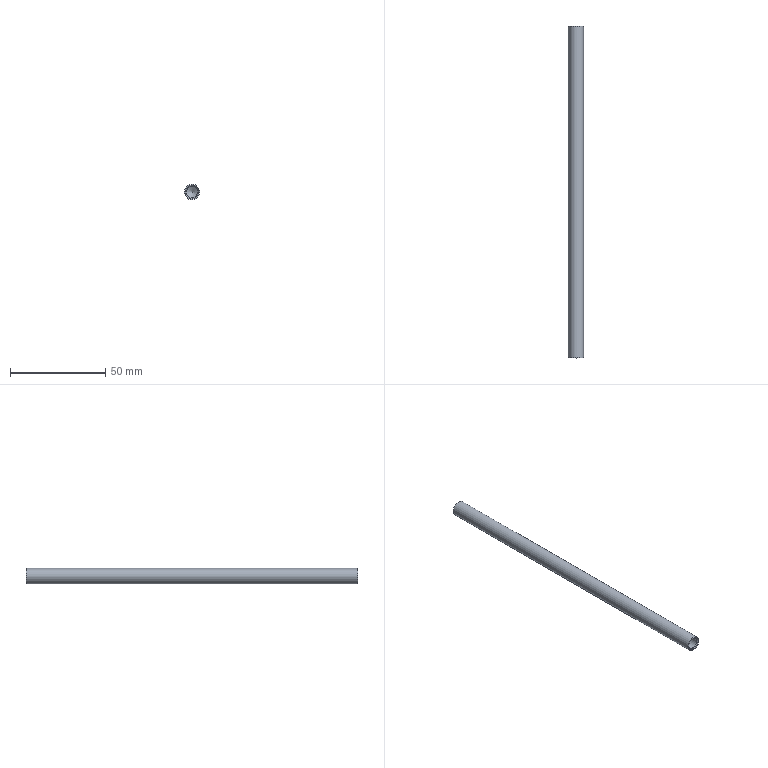Component | NX | CONNECTING_ROD_2 | 1 solid | 9 faces | box 8 x 174 x 8 mm | volume 7746 mm3 | cone 4 | cylinder 3 | plane 2 | commonest cylinder face diameters 6 x2 8 x1
STEP:
#1=CARTESIAN_POINT('',(0.,0.,0.));
#2=DIRECTION('',(0.,0.,1.));
#3=DIRECTION('',(1.,0.,0.));
#4=AXIS2_PLACEMENT_3D('',#1,#2,#3);
#5=CARTESIAN_POINT('',(-245.053,87.,124.782));
#6=VERTEX_POINT('',#5);
#7=CARTESIAN_POINT('',(-248.225,87.,123.303));
#8=DIRECTION('',(0.,-1.,0.));
#9=DIRECTION('',(0.9063,0.,0.4226));
#10=AXIS2_PLACEMENT_3D('',#7,#8,#9);
#11=CIRCLE('',#10,3.5);
#12=CARTESIAN_POINT('',(-248.225,87.,123.303));
#13=DIRECTION('',(0.,1.,0.));
#14=DIRECTION('',(0.9063,0.,0.4226));
#15=AXIS2_PLACEMENT_3D('',#12,#13,#14);
#16=PLANE('',#15);
#17=CARTESIAN_POINT('',(3.5,0.));
#18=CARTESIAN_POINT('',(3.5,-6.062));
#19=CARTESIAN_POINT('',(-1.75,-3.031));
#20=CARTESIAN_POINT('',(-7.,-0.));
#21=CARTESIAN_POINT('',(-1.75,3.031));
#22=CARTESIAN_POINT('',(3.5,6.062));
#23=CARTESIAN_POINT('',(3.5,0.));
#24=(BOUNDED_CURVE()B_SPLINE_CURVE(2,(#17,#18,#19,#20,#21,#22,#23),.UNSPECIFIED.,.T.,.F.)B_SPLINE_CURVE_WITH_KNOTS((1,2,2,2,2,1),(-2.094,0.,2.094,4.189,6.283,8.378),.UNSPECIFIED.)CURVE()GEOMETRIC_REPRESENTATION_ITEM()RATIONAL_B_SPLINE_CURVE((1.,0.5,1.,0.5,1.,0.5,1.))REPRESENTATION_ITEM(''));
#25=(GEOMETRIC_REPRESENTATION_CONTEXT(2)PARAMETRIC_REPRESENTATION_CONTEXT()REPRESENTATION_CONTEXT('',''));
#26=DEFINITIONAL_REPRESENTATION('',(#24),#25);
#27=PCURVE('',#16,#26);
#28=CARTESIAN_POINT('',(-248.225,87.,123.303));
#29=DIRECTION('',(0.,1.,0.));
#30=DIRECTION('',(0.9063,0.,0.4226));
#31=AXIS2_PLACEMENT_3D('',#28,#29,#30);
#32=CONICAL_SURFACE('',#31,3.5,0.7854);
#33=CARTESIAN_POINT('',(6.283,0.));
#34=DIRECTION('',(-1.,0.));
#35=VECTOR('',#34,1.);
#36=LINE('',#33,#35);
#37=(GEOMETRIC_REPRESENTATION_CONTEXT(2)PARAMETRIC_REPRESENTATION_CONTEXT()REPRESENTATION_CONTEXT('',''));
#38=DEFINITIONAL_REPRESENTATION('',(#36),#37);
#39=PCURVE('',#32,#38);
#40=SURFACE_CURVE('',#11,(#27,#39),.PCURVE_S1.);
#41=EDGE_CURVE('',#6,#6,#40,.T.);
#42=ORIENTED_EDGE('',*,*,#41,.T.);
#43=EDGE_LOOP('',(#42));
#44=FACE_BOUND('',#43,.T.);
#45=CARTESIAN_POINT('',(-244.6,87.,124.993));
#46=VERTEX_POINT('',#45);
#47=CARTESIAN_POINT('',(-248.225,87.,123.303));
#48=DIRECTION('',(0.,-1.,0.));
#49=DIRECTION('',(0.9063,0.,0.4226));
#50=AXIS2_PLACEMENT_3D('',#47,#48,#49);
#51=CIRCLE('',#50,4.);
#52=CARTESIAN_POINT('',(4.,-0.));
#53=CARTESIAN_POINT('',(4.,-6.928));
#54=CARTESIAN_POINT('',(-2.,-3.464));
#55=CARTESIAN_POINT('',(-8.,0.));
#56=CARTESIAN_POINT('',(-2.,3.464));
#57=CARTESIAN_POINT('',(4.,6.928));
#58=CARTESIAN_POINT('',(4.,-0.));
#59=(BOUNDED_CURVE()B_SPLINE_CURVE(2,(#52,#53,#54,#55,#56,#57,#58),.UNSPECIFIED.,.T.,.F.)B_SPLINE_CURVE_WITH_KNOTS((1,2,2,2,2,1),(-2.094,0.,2.094,4.189,6.283,8.378),.UNSPECIFIED.)CURVE()GEOMETRIC_REPRESENTATION_ITEM()RATIONAL_B_SPLINE_CURVE((1.,0.5,1.,0.5,1.,0.5,1.))REPRESENTATION_ITEM(''));
#60=(GEOMETRIC_REPRESENTATION_CONTEXT(2)PARAMETRIC_REPRESENTATION_CONTEXT()REPRESENTATION_CONTEXT('',''));
#61=DEFINITIONAL_REPRESENTATION('',(#59),#60);
#62=PCURVE('',#16,#61);
#63=CARTESIAN_POINT('',(-248.225,-87.,123.303));
#64=DIRECTION('',(0.,1.,0.));
#65=DIRECTION('',(0.9063,0.,0.4226));
#66=AXIS2_PLACEMENT_3D('',#63,#64,#65);
#67=CYLINDRICAL_SURFACE('',#66,4.);
#68=CARTESIAN_POINT('',(6.283,174.));
#69=DIRECTION('',(-1.,0.));
#70=VECTOR('',#69,1.);
#71=LINE('',#68,#70);
#72=(GEOMETRIC_REPRESENTATION_CONTEXT(2)PARAMETRIC_REPRESENTATION_CONTEXT()REPRESENTATION_CONTEXT('',''));
#73=DEFINITIONAL_REPRESENTATION('',(#71),#72);
#74=PCURVE('',#67,#73);
#75=SURFACE_CURVE('',#51,(#62,#74),.PCURVE_S1.);
#76=EDGE_CURVE('',#46,#46,#75,.T.);
#77=ORIENTED_EDGE('',*,*,#76,.F.);
#78=EDGE_LOOP('',(#77));
#79=FACE_BOUND('',#78,.T.);
#80=ADVANCED_FACE('',(#44,#79),#16,.T.);
#81=CARTESIAN_POINT('',(-251.397,-87.,121.824));
#82=VERTEX_POINT('',#81);
#83=CARTESIAN_POINT('',(-248.225,-87.,123.303));
#84=DIRECTION('',(0.,1.,0.));
#85=DIRECTION('',(-0.9063,0.,-0.4226));
#86=AXIS2_PLACEMENT_3D('',#83,#84,#85);
#87=CIRCLE('',#86,3.5);
#88=CARTESIAN_POINT('',(-248.225,-87.,123.303));
#89=DIRECTION('',(0.,-1.,0.));
#90=DIRECTION('',(-0.9063,0.,-0.4226));
#91=AXIS2_PLACEMENT_3D('',#88,#89,#90);
#92=PLANE('',#91);
#93=CARTESIAN_POINT('',(3.5,-0.));
#94=CARTESIAN_POINT('',(3.5,-6.062));
#95=CARTESIAN_POINT('',(-1.75,-3.031));
#96=CARTESIAN_POINT('',(-7.,0.));
#97=CARTESIAN_POINT('',(-1.75,3.031));
#98=CARTESIAN_POINT('',(3.5,6.062));
#99=CARTESIAN_POINT('',(3.5,-0.));
#100=(BOUNDED_CURVE()B_SPLINE_CURVE(2,(#93,#94,#95,#96,#97,#98,#99),.UNSPECIFIED.,.T.,.F.)B_SPLINE_CURVE_WITH_KNOTS((1,2,2,2,2,1),(-2.094,0.,2.094,4.189,6.283,8.378),.UNSPECIFIED.)CURVE()GEOMETRIC_REPRESENTATION_ITEM()RATIONAL_B_SPLINE_CURVE((1.,0.5,1.,0.5,1.,0.5,1.))REPRESENTATION_ITEM(''));
#101=(GEOMETRIC_REPRESENTATION_CONTEXT(2)PARAMETRIC_REPRESENTATION_CONTEXT()REPRESENTATION_CONTEXT('',''));
#102=DEFINITIONAL_REPRESENTATION('',(#100),#101);
#103=PCURVE('',#92,#102);
#104=CARTESIAN_POINT('',(-248.225,-87.,123.303));
#105=DIRECTION('',(0.,-1.,0.));
#106=DIRECTION('',(-0.9063,0.,-0.4226));
#107=AXIS2_PLACEMENT_3D('',#104,#105,#106);
#108=CONICAL_SURFACE('',#107,3.5,0.7854);
#109=CARTESIAN_POINT('',(6.283,0.));
#110=DIRECTION('',(-1.,0.));
#111=VECTOR('',#110,1.);
#112=LINE('',#109,#111);
#113=(GEOMETRIC_REPRESENTATION_CONTEXT(2)PARAMETRIC_REPRESENTATION_CONTEXT()REPRESENTATION_CONTEXT('',''));
#114=DEFINITIONAL_REPRESENTATION('',(#112),#113);
#115=PCURVE('',#108,#114);
#116=SURFACE_CURVE('',#87,(#103,#115),.PCURVE_S1.);
#117=EDGE_CURVE('',#82,#82,#116,.T.);
#118=ORIENTED_EDGE('',*,*,#117,.T.);
#119=EDGE_LOOP('',(#118));
#120=FACE_BOUND('',#119,.T.);
#121=CARTESIAN_POINT('',(-244.6,-87.,124.993));
#122=VERTEX_POINT('',#121);
#123=CARTESIAN_POINT('',(-248.225,-87.,123.303));
#124=DIRECTION('',(0.,1.,0.));
#125=DIRECTION('',(0.9063,0.,0.4226));
#126=AXIS2_PLACEMENT_3D('',#123,#124,#125);
#127=CIRCLE('',#126,4.);
#128=CARTESIAN_POINT('',(-4.,-0.));
#129=CARTESIAN_POINT('',(-4.,6.928));
#130=CARTESIAN_POINT('',(2.,3.464));
#131=CARTESIAN_POINT('',(8.,0.));
#132=CARTESIAN_POINT('',(2.,-3.464));
#133=CARTESIAN_POINT('',(-4.,-6.928));
#134=CARTESIAN_POINT('',(-4.,-0.));
#135=(BOUNDED_CURVE()B_SPLINE_CURVE(2,(#128,#129,#130,#131,#132,#133,#134),.UNSPECIFIED.,.T.,.F.)B_SPLINE_CURVE_WITH_KNOTS((1,2,2,2,2,1),(-2.094,0.,2.094,4.189,6.283,8.378),.UNSPECIFIED.)CURVE()GEOMETRIC_REPRESENTATION_ITEM()RATIONAL_B_SPLINE_CURVE((1.,0.5,1.,0.5,1.,0.5,1.))REPRESENTATION_ITEM(''));
#136=(GEOMETRIC_REPRESENTATION_CONTEXT(2)PARAMETRIC_REPRESENTATION_CONTEXT()REPRESENTATION_CONTEXT('',''));
#137=DEFINITIONAL_REPRESENTATION('',(#135),#136);
#138=PCURVE('',#92,#137);
#139=CARTESIAN_POINT('',(0.,0.));
#140=DIRECTION('',(1.,0.));
#141=VECTOR('',#140,1.);
#142=LINE('',#139,#141);
#143=(GEOMETRIC_REPRESENTATION_CONTEXT(2)PARAMETRIC_REPRESENTATION_CONTEXT()REPRESENTATION_CONTEXT('',''));
#144=DEFINITIONAL_REPRESENTATION('',(#142),#143);
#145=PCURVE('',#67,#144);
#146=SURFACE_CURVE('',#127,(#138,#145),.PCURVE_S1.);
#147=EDGE_CURVE('',#122,#122,#146,.T.);
#148=ORIENTED_EDGE('',*,*,#147,.F.);
#149=EDGE_LOOP('',(#148));
#150=FACE_BOUND('',#149,.T.);
#151=ADVANCED_FACE('',(#120,#150),#92,.T.);
#152=ORIENTED_EDGE('',*,*,#76,.T.);
#153=CARTESIAN_POINT('',(-244.6,-87.,124.993));
#154=CARTESIAN_POINT('',(-244.6,87.,124.993));
#155=B_SPLINE_CURVE_WITH_KNOTS('',1,(#153,#154),.UNSPECIFIED.,.F.,.F.,(2,2),(0.,174.),.PIECEWISE_BEZIER_KNOTS.);
#156=CARTESIAN_POINT('',(0.,0.));
#157=DIRECTION('',(0.,1.));
#158=VECTOR('',#157,1.);
#159=LINE('',#156,#158);
#160=(GEOMETRIC_REPRESENTATION_CONTEXT(2)PARAMETRIC_REPRESENTATION_CONTEXT()REPRESENTATION_CONTEXT('',''));
#161=DEFINITIONAL_REPRESENTATION('',(#159),#160);
#162=PCURVE('',#67,#161);
#163=CARTESIAN_POINT('',(6.283,0.));
#164=DIRECTION('',(0.,1.));
#165=VECTOR('',#164,1.);
#166=LINE('',#163,#165);
#167=(GEOMETRIC_REPRESENTATION_CONTEXT(2)PARAMETRIC_REPRESENTATION_CONTEXT()REPRESENTATION_CONTEXT('',''));
#168=DEFINITIONAL_REPRESENTATION('',(#166),#167);
#169=PCURVE('',#67,#168);
#170=SEAM_CURVE('',#155,(#162,#169),.PCURVE_S1.);
#171=EDGE_CURVE('',#122,#46,#170,.T.);
#172=ORIENTED_EDGE('',*,*,#171,.F.);
#173=ORIENTED_EDGE('',*,*,#147,.T.);
#174=ORIENTED_EDGE('',*,*,#171,.T.);
#175=EDGE_LOOP('',(#152,#172,#173,#174));
#176=FACE_BOUND('',#175,.T.);
#177=ADVANCED_FACE('',(#176),#67,.T.);
#178=CARTESIAN_POINT('',(-245.506,70.,124.571));
#179=VERTEX_POINT('',#178);
#180=CARTESIAN_POINT('',(-250.944,70.,122.035));
#181=VERTEX_POINT('',#180);
#182=CARTESIAN_POINT('',(-248.225,70.,123.303));
#183=DIRECTION('',(0.,1.,0.));
#184=DIRECTION('',(-0.9063,0.,-0.4226));
#185=AXIS2_PLACEMENT_3D('',#182,#183,#184);
#186=CIRCLE('',#185,3.);
#187=CARTESIAN_POINT('',(-248.225,70.,123.303));
#188=DIRECTION('',(0.,1.,0.));
#189=DIRECTION('',(0.9063,0.,0.4226));
#190=AXIS2_PLACEMENT_3D('',#187,#188,#189);
#191=CONICAL_SURFACE('',#190,3.,1.03);
#192=CARTESIAN_POINT('',(-3.142,-0.));
#193=DIRECTION('',(1.,0.));
#194=VECTOR('',#193,1.);
#195=LINE('',#192,#194);
#196=(GEOMETRIC_REPRESENTATION_CONTEXT(2)PARAMETRIC_REPRESENTATION_CONTEXT()REPRESENTATION_CONTEXT('',''));
#197=DEFINITIONAL_REPRESENTATION('',(#195),#196);
#198=PCURVE('',#191,#197);
#199=CARTESIAN_POINT('',(-248.225,87.,123.303));
#200=DIRECTION('',(0.,-1.,0.));
#201=DIRECTION('',(-0.9063,0.,-0.4226));
#202=AXIS2_PLACEMENT_3D('',#199,#200,#201);
#203=CYLINDRICAL_SURFACE('',#202,3.);
#204=CARTESIAN_POINT('',(12.566,17.));
#205=DIRECTION('',(-1.,0.));
#206=VECTOR('',#205,1.);
#207=LINE('',#204,#206);
#208=(GEOMETRIC_REPRESENTATION_CONTEXT(2)PARAMETRIC_REPRESENTATION_CONTEXT()REPRESENTATION_CONTEXT('',''));
#209=DEFINITIONAL_REPRESENTATION('',(#207),#208);
#210=PCURVE('',#203,#209);
#211=SURFACE_CURVE('',#186,(#198,#210),.PCURVE_S1.);
#212=EDGE_CURVE('',#179,#181,#211,.T.);
#213=ORIENTED_EDGE('',*,*,#212,.F.);
#214=CARTESIAN_POINT('',(-248.225,68.197,123.303));
#215=VERTEX_POINT('',#214);
#216=CARTESIAN_POINT('',(-248.225,68.197,123.303));
#217=CARTESIAN_POINT('',(-245.506,70.,124.571));
#218=B_SPLINE_CURVE_WITH_KNOTS('',1,(#216,#217),.UNSPECIFIED.,.F.,.F.,(2,2),(-3.5,-0.),.PIECEWISE_BEZIER_KNOTS.);
#219=CARTESIAN_POINT('',(0.,0.));
#220=DIRECTION('',(0.,1.));
#221=VECTOR('',#220,1.);
#222=LINE('',#219,#221);
#223=(GEOMETRIC_REPRESENTATION_CONTEXT(2)PARAMETRIC_REPRESENTATION_CONTEXT()REPRESENTATION_CONTEXT('',''));
#224=DEFINITIONAL_REPRESENTATION('',(#222),#223);
#225=PCURVE('',#191,#224);
#226=CARTESIAN_POINT('',(6.283,0.));
#227=DIRECTION('',(0.,1.));
#228=VECTOR('',#227,1.);
#229=LINE('',#226,#228);
#230=(GEOMETRIC_REPRESENTATION_CONTEXT(2)PARAMETRIC_REPRESENTATION_CONTEXT()REPRESENTATION_CONTEXT('',''));
#231=DEFINITIONAL_REPRESENTATION('',(#229),#230);
#232=PCURVE('',#191,#231);
#233=SEAM_CURVE('',#218,(#225,#232),.PCURVE_S1.);
#234=EDGE_CURVE('',#215,#179,#233,.T.);
#235=ORIENTED_EDGE('',*,*,#234,.F.);
#236=ORIENTED_EDGE('',*,*,#234,.T.);
#237=CARTESIAN_POINT('',(-248.225,70.,123.303));
#238=DIRECTION('',(0.,1.,0.));
#239=DIRECTION('',(-0.9063,0.,-0.4226));
#240=AXIS2_PLACEMENT_3D('',#237,#238,#239);
#241=CIRCLE('',#240,3.);
#242=CARTESIAN_POINT('',(3.142,-0.));
#243=DIRECTION('',(1.,0.));
#244=VECTOR('',#243,1.);
#245=LINE('',#242,#244);
#246=(GEOMETRIC_REPRESENTATION_CONTEXT(2)PARAMETRIC_REPRESENTATION_CONTEXT()REPRESENTATION_CONTEXT('',''));
#247=DEFINITIONAL_REPRESENTATION('',(#245),#246);
#248=PCURVE('',#191,#247);
#249=CARTESIAN_POINT('',(6.283,17.));
#250=DIRECTION('',(-1.,0.));
#251=VECTOR('',#250,1.);
#252=LINE('',#249,#251);
#253=(GEOMETRIC_REPRESENTATION_CONTEXT(2)PARAMETRIC_REPRESENTATION_CONTEXT()REPRESENTATION_CONTEXT('',''));
#254=DEFINITIONAL_REPRESENTATION('',(#252),#253);
#255=PCURVE('',#203,#254);
#256=SURFACE_CURVE('',#241,(#248,#255),.PCURVE_S1.);
#257=EDGE_CURVE('',#181,#179,#256,.T.);
#258=ORIENTED_EDGE('',*,*,#257,.F.);
#259=EDGE_LOOP('',(#213,#235,#236,#258));
#260=FACE_BOUND('',#259,.F.);
#261=ADVANCED_FACE('',(#260),#191,.F.);
#262=CARTESIAN_POINT('',(-245.506,86.5,124.571));
#263=VERTEX_POINT('',#262);
#264=CARTESIAN_POINT('',(-248.225,86.5,123.303));
#265=DIRECTION('',(0.,1.,0.));
#266=DIRECTION('',(0.9063,0.,0.4226));
#267=AXIS2_PLACEMENT_3D('',#264,#265,#266);
#268=CIRCLE('',#267,3.);
#269=CARTESIAN_POINT('',(9.425,0.5));
#270=DIRECTION('',(-1.,0.));
#271=VECTOR('',#270,1.);
#272=LINE('',#269,#271);
#273=(GEOMETRIC_REPRESENTATION_CONTEXT(2)PARAMETRIC_REPRESENTATION_CONTEXT()REPRESENTATION_CONTEXT('',''));
#274=DEFINITIONAL_REPRESENTATION('',(#272),#273);
#275=PCURVE('',#203,#274);
#276=CARTESIAN_POINT('',(0.,-0.5));
#277=DIRECTION('',(1.,0.));
#278=VECTOR('',#277,1.);
#279=LINE('',#276,#278);
#280=(GEOMETRIC_REPRESENTATION_CONTEXT(2)PARAMETRIC_REPRESENTATION_CONTEXT()REPRESENTATION_CONTEXT('',''));
#281=DEFINITIONAL_REPRESENTATION('',(#279),#280);
#282=PCURVE('',#32,#281);
#283=SURFACE_CURVE('',#268,(#275,#282),.PCURVE_S1.);
#284=EDGE_CURVE('',#263,#263,#283,.T.);
#285=ORIENTED_EDGE('',*,*,#284,.F.);
#286=CARTESIAN_POINT('',(-245.506,86.5,124.571));
#287=CARTESIAN_POINT('',(-245.506,70.,124.571));
#288=B_SPLINE_CURVE_WITH_KNOTS('',1,(#286,#287),.UNSPECIFIED.,.F.,.F.,(2,2),(0.5,17.),.PIECEWISE_BEZIER_KNOTS.);
#289=CARTESIAN_POINT('',(9.425,0.));
#290=DIRECTION('',(0.,1.));
#291=VECTOR('',#290,1.);
#292=LINE('',#289,#291);
#293=(GEOMETRIC_REPRESENTATION_CONTEXT(2)PARAMETRIC_REPRESENTATION_CONTEXT()REPRESENTATION_CONTEXT('',''));
#294=DEFINITIONAL_REPRESENTATION('',(#292),#293);
#295=PCURVE('',#203,#294);
#296=CARTESIAN_POINT('',(3.142,0.));
#297=DIRECTION('',(0.,1.));
#298=VECTOR('',#297,1.);
#299=LINE('',#296,#298);
#300=(GEOMETRIC_REPRESENTATION_CONTEXT(2)PARAMETRIC_REPRESENTATION_CONTEXT()REPRESENTATION_CONTEXT('',''));
#301=DEFINITIONAL_REPRESENTATION('',(#299),#300);
#302=PCURVE('',#203,#301);
#303=SEAM_CURVE('',#288,(#295,#302),.PCURVE_S1.);
#304=EDGE_CURVE('',#263,#179,#303,.T.);
#305=ORIENTED_EDGE('',*,*,#304,.T.);
#306=ORIENTED_EDGE('',*,*,#212,.T.);
#307=ORIENTED_EDGE('',*,*,#257,.T.);
#308=ORIENTED_EDGE('',*,*,#304,.F.);
#309=EDGE_LOOP('',(#285,#305,#306,#307,#308));
#310=FACE_BOUND('',#309,.F.);
#311=ADVANCED_FACE('',(#310),#203,.F.);
#312=ORIENTED_EDGE('',*,*,#284,.T.);
#313=CARTESIAN_POINT('',(-245.506,86.5,124.571));
#314=CARTESIAN_POINT('',(-245.053,87.,124.782));
#315=B_SPLINE_CURVE_WITH_KNOTS('',1,(#313,#314),.UNSPECIFIED.,.F.,.F.,(2,2),(-0.7071,0.),.PIECEWISE_BEZIER_KNOTS.);
#316=CARTESIAN_POINT('',(6.283,0.));
#317=DIRECTION('',(0.,1.));
#318=VECTOR('',#317,1.);
#319=LINE('',#316,#318);
#320=(GEOMETRIC_REPRESENTATION_CONTEXT(2)PARAMETRIC_REPRESENTATION_CONTEXT()REPRESENTATION_CONTEXT('',''));
#321=DEFINITIONAL_REPRESENTATION('',(#319),#320);
#322=PCURVE('',#32,#321);
#323=CARTESIAN_POINT('',(0.,0.));
#324=DIRECTION('',(0.,1.));
#325=VECTOR('',#324,1.);
#326=LINE('',#323,#325);
#327=(GEOMETRIC_REPRESENTATION_CONTEXT(2)PARAMETRIC_REPRESENTATION_CONTEXT()REPRESENTATION_CONTEXT('',''));
#328=DEFINITIONAL_REPRESENTATION('',(#326),#327);
#329=PCURVE('',#32,#328);
#330=SEAM_CURVE('',#315,(#322,#329),.PCURVE_S1.);
#331=EDGE_CURVE('',#263,#6,#330,.T.);
#332=ORIENTED_EDGE('',*,*,#331,.T.);
#333=ORIENTED_EDGE('',*,*,#41,.T.);
#334=ORIENTED_EDGE('',*,*,#331,.F.);
#335=EDGE_LOOP('',(#312,#332,#333,#334));
#336=FACE_BOUND('',#335,.F.);
#337=ADVANCED_FACE('',(#336),#32,.F.);
#338=CARTESIAN_POINT('',(-250.944,-70.,122.035));
#339=VERTEX_POINT('',#338);
#340=CARTESIAN_POINT('',(-245.506,-70.,124.571));
#341=VERTEX_POINT('',#340);
#342=CARTESIAN_POINT('',(-248.225,-70.,123.303));
#343=DIRECTION('',(0.,-1.,0.));
#344=DIRECTION('',(0.9063,0.,0.4226));
#345=AXIS2_PLACEMENT_3D('',#342,#343,#344);
#346=CIRCLE('',#345,3.);
#347=CARTESIAN_POINT('',(-248.225,-70.,123.303));
#348=DIRECTION('',(0.,-1.,0.));
#349=DIRECTION('',(-0.9063,0.,-0.4226));
#350=AXIS2_PLACEMENT_3D('',#347,#348,#349);
#351=CONICAL_SURFACE('',#350,3.,1.03);
#352=CARTESIAN_POINT('',(-3.142,0.));
#353=DIRECTION('',(1.,0.));
#354=VECTOR('',#353,1.);
#355=LINE('',#352,#354);
#356=(GEOMETRIC_REPRESENTATION_CONTEXT(2)PARAMETRIC_REPRESENTATION_CONTEXT()REPRESENTATION_CONTEXT('',''));
#357=DEFINITIONAL_REPRESENTATION('',(#355),#356);
#358=PCURVE('',#351,#357);
#359=CARTESIAN_POINT('',(-248.225,-87.,123.303));
#360=DIRECTION('',(0.,1.,0.));
#361=DIRECTION('',(0.9063,0.,0.4226));
#362=AXIS2_PLACEMENT_3D('',#359,#360,#361);
#363=CYLINDRICAL_SURFACE('',#362,3.);
#364=CARTESIAN_POINT('',(12.566,17.));
#365=DIRECTION('',(-1.,0.));
#366=VECTOR('',#365,1.);
#367=LINE('',#364,#366);
#368=(GEOMETRIC_REPRESENTATION_CONTEXT(2)PARAMETRIC_REPRESENTATION_CONTEXT()REPRESENTATION_CONTEXT('',''));
#369=DEFINITIONAL_REPRESENTATION('',(#367),#368);
#370=PCURVE('',#363,#369);
#371=SURFACE_CURVE('',#346,(#358,#370),.PCURVE_S1.);
#372=EDGE_CURVE('',#339,#341,#371,.T.);
#373=ORIENTED_EDGE('',*,*,#372,.F.);
#374=CARTESIAN_POINT('',(-248.225,-68.197,123.303));
#375=VERTEX_POINT('',#374);
#376=CARTESIAN_POINT('',(-248.225,-68.197,123.303));
#377=CARTESIAN_POINT('',(-250.944,-70.,122.035));
#378=B_SPLINE_CURVE_WITH_KNOTS('',1,(#376,#377),.UNSPECIFIED.,.F.,.F.,(2,2),(-3.5,0.),.PIECEWISE_BEZIER_KNOTS.);
#379=CARTESIAN_POINT('',(0.,0.));
#380=DIRECTION('',(0.,1.));
#381=VECTOR('',#380,1.);
#382=LINE('',#379,#381);
#383=(GEOMETRIC_REPRESENTATION_CONTEXT(2)PARAMETRIC_REPRESENTATION_CONTEXT()REPRESENTATION_CONTEXT('',''));
#384=DEFINITIONAL_REPRESENTATION('',(#382),#383);
#385=PCURVE('',#351,#384);
#386=CARTESIAN_POINT('',(6.283,0.));
#387=DIRECTION('',(0.,1.));
#388=VECTOR('',#387,1.);
#389=LINE('',#386,#388);
#390=(GEOMETRIC_REPRESENTATION_CONTEXT(2)PARAMETRIC_REPRESENTATION_CONTEXT()REPRESENTATION_CONTEXT('',''));
#391=DEFINITIONAL_REPRESENTATION('',(#389),#390);
#392=PCURVE('',#351,#391);
#393=SEAM_CURVE('',#378,(#385,#392),.PCURVE_S1.);
#394=EDGE_CURVE('',#375,#339,#393,.T.);
#395=ORIENTED_EDGE('',*,*,#394,.F.);
#396=ORIENTED_EDGE('',*,*,#394,.T.);
#397=CARTESIAN_POINT('',(-248.225,-70.,123.303));
#398=DIRECTION('',(0.,-1.,0.));
#399=DIRECTION('',(0.9063,0.,0.4226));
#400=AXIS2_PLACEMENT_3D('',#397,#398,#399);
#401=CIRCLE('',#400,3.);
#402=CARTESIAN_POINT('',(3.142,0.));
#403=DIRECTION('',(1.,0.));
#404=VECTOR('',#403,1.);
#405=LINE('',#402,#404);
#406=(GEOMETRIC_REPRESENTATION_CONTEXT(2)PARAMETRIC_REPRESENTATION_CONTEXT()REPRESENTATION_CONTEXT('',''));
#407=DEFINITIONAL_REPRESENTATION('',(#405),#406);
#408=PCURVE('',#351,#407);
#409=CARTESIAN_POINT('',(6.283,17.));
#410=DIRECTION('',(-1.,0.));
#411=VECTOR('',#410,1.);
#412=LINE('',#409,#411);
#413=(GEOMETRIC_REPRESENTATION_CONTEXT(2)PARAMETRIC_REPRESENTATION_CONTEXT()REPRESENTATION_CONTEXT('',''));
#414=DEFINITIONAL_REPRESENTATION('',(#412),#413);
#415=PCURVE('',#363,#414);
#416=SURFACE_CURVE('',#401,(#408,#415),.PCURVE_S1.);
#417=EDGE_CURVE('',#341,#339,#416,.T.);
#418=ORIENTED_EDGE('',*,*,#417,.F.);
#419=EDGE_LOOP('',(#373,#395,#396,#418));
#420=FACE_BOUND('',#419,.F.);
#421=ADVANCED_FACE('',(#420),#351,.F.);
#422=CARTESIAN_POINT('',(-250.944,-86.5,122.035));
#423=VERTEX_POINT('',#422);
#424=CARTESIAN_POINT('',(-248.225,-86.5,123.303));
#425=DIRECTION('',(0.,-1.,0.));
#426=DIRECTION('',(-0.9063,0.,-0.4226));
#427=AXIS2_PLACEMENT_3D('',#424,#425,#426);
#428=CIRCLE('',#427,3.);
#429=CARTESIAN_POINT('',(9.425,0.5));
#430=DIRECTION('',(-1.,0.));
#431=VECTOR('',#430,1.);
#432=LINE('',#429,#431);
#433=(GEOMETRIC_REPRESENTATION_CONTEXT(2)PARAMETRIC_REPRESENTATION_CONTEXT()REPRESENTATION_CONTEXT('',''));
#434=DEFINITIONAL_REPRESENTATION('',(#432),#433);
#435=PCURVE('',#363,#434);
#436=CARTESIAN_POINT('',(0.,-0.5));
#437=DIRECTION('',(1.,0.));
#438=VECTOR('',#437,1.);
#439=LINE('',#436,#438);
#440=(GEOMETRIC_REPRESENTATION_CONTEXT(2)PARAMETRIC_REPRESENTATION_CONTEXT()REPRESENTATION_CONTEXT('',''));
#441=DEFINITIONAL_REPRESENTATION('',(#439),#440);
#442=PCURVE('',#108,#441);
#443=SURFACE_CURVE('',#428,(#435,#442),.PCURVE_S1.);
#444=EDGE_CURVE('',#423,#423,#443,.T.);
#445=ORIENTED_EDGE('',*,*,#444,.F.);
#446=CARTESIAN_POINT('',(-250.944,-86.5,122.035));
#447=CARTESIAN_POINT('',(-250.944,-70.,122.035));
#448=B_SPLINE_CURVE_WITH_KNOTS('',1,(#446,#447),.UNSPECIFIED.,.F.,.F.,(2,2),(0.5,17.),.PIECEWISE_BEZIER_KNOTS.);
#449=CARTESIAN_POINT('',(9.425,0.));
#450=DIRECTION('',(0.,1.));
#451=VECTOR('',#450,1.);
#452=LINE('',#449,#451);
#453=(GEOMETRIC_REPRESENTATION_CONTEXT(2)PARAMETRIC_REPRESENTATION_CONTEXT()REPRESENTATION_CONTEXT('',''));
#454=DEFINITIONAL_REPRESENTATION('',(#452),#453);
#455=PCURVE('',#363,#454);
#456=CARTESIAN_POINT('',(3.142,0.));
#457=DIRECTION('',(0.,1.));
#458=VECTOR('',#457,1.);
#459=LINE('',#456,#458);
#460=(GEOMETRIC_REPRESENTATION_CONTEXT(2)PARAMETRIC_REPRESENTATION_CONTEXT()REPRESENTATION_CONTEXT('',''));
#461=DEFINITIONAL_REPRESENTATION('',(#459),#460);
#462=PCURVE('',#363,#461);
#463=SEAM_CURVE('',#448,(#455,#462),.PCURVE_S1.);
#464=EDGE_CURVE('',#423,#339,#463,.T.);
#465=ORIENTED_EDGE('',*,*,#464,.T.);
#466=ORIENTED_EDGE('',*,*,#372,.T.);
#467=ORIENTED_EDGE('',*,*,#417,.T.);
#468=ORIENTED_EDGE('',*,*,#464,.F.);
#469=EDGE_LOOP('',(#445,#465,#466,#467,#468));
#470=FACE_BOUND('',#469,.F.);
#471=ADVANCED_FACE('',(#470),#363,.F.);
#472=ORIENTED_EDGE('',*,*,#444,.T.);
#473=CARTESIAN_POINT('',(-250.944,-86.5,122.035));
#474=CARTESIAN_POINT('',(-251.397,-87.,121.824));
#475=B_SPLINE_CURVE_WITH_KNOTS('',1,(#473,#474),.UNSPECIFIED.,.F.,.F.,(2,2),(-0.7071,0.),.PIECEWISE_BEZIER_KNOTS.);
#476=CARTESIAN_POINT('',(6.283,0.));
#477=DIRECTION('',(0.,1.));
#478=VECTOR('',#477,1.);
#479=LINE('',#476,#478);
#480=(GEOMETRIC_REPRESENTATION_CONTEXT(2)PARAMETRIC_REPRESENTATION_CONTEXT()REPRESENTATION_CONTEXT('',''));
#481=DEFINITIONAL_REPRESENTATION('',(#479),#480);
#482=PCURVE('',#108,#481);
#483=CARTESIAN_POINT('',(0.,0.));
#484=DIRECTION('',(0.,1.));
#485=VECTOR('',#484,1.);
#486=LINE('',#483,#485);
#487=(GEOMETRIC_REPRESENTATION_CONTEXT(2)PARAMETRIC_REPRESENTATION_CONTEXT()REPRESENTATION_CONTEXT('',''));
#488=DEFINITIONAL_REPRESENTATION('',(#486),#487);
#489=PCURVE('',#108,#488);
#490=SEAM_CURVE('',#475,(#482,#489),.PCURVE_S1.);
#491=EDGE_CURVE('',#423,#82,#490,.T.);
#492=ORIENTED_EDGE('',*,*,#491,.T.);
#493=ORIENTED_EDGE('',*,*,#117,.T.);
#494=ORIENTED_EDGE('',*,*,#491,.F.);
#495=EDGE_LOOP('',(#472,#492,#493,#494));
#496=FACE_BOUND('',#495,.F.);
#497=ADVANCED_FACE('',(#496),#108,.F.);
#498=CLOSED_SHELL('',(#80,#151,#177,#261,#311,#337,#421,#471,#497));
#499=MANIFOLD_SOLID_BREP('',#498);
#500=(LENGTH_UNIT()NAMED_UNIT(*)SI_UNIT(.MILLI.,.METRE.));
#501=UNCERTAINTY_MEASURE_WITH_UNIT(LENGTH_MEASURE(0.00001),#500,'','');
#502=(NAMED_UNIT(*)PLANE_ANGLE_UNIT()SI_UNIT($,.RADIAN.));
#503=(NAMED_UNIT(*)SI_UNIT($,.STERADIAN.)SOLID_ANGLE_UNIT());
#504=(GEOMETRIC_REPRESENTATION_CONTEXT(3)GLOBAL_UNCERTAINTY_ASSIGNED_CONTEXT((#501))GLOBAL_UNIT_ASSIGNED_CONTEXT((#500,#502,#503))REPRESENTATION_CONTEXT('',''));
#505=ADVANCED_BREP_SHAPE_REPRESENTATION('',(#4,#499),#504);